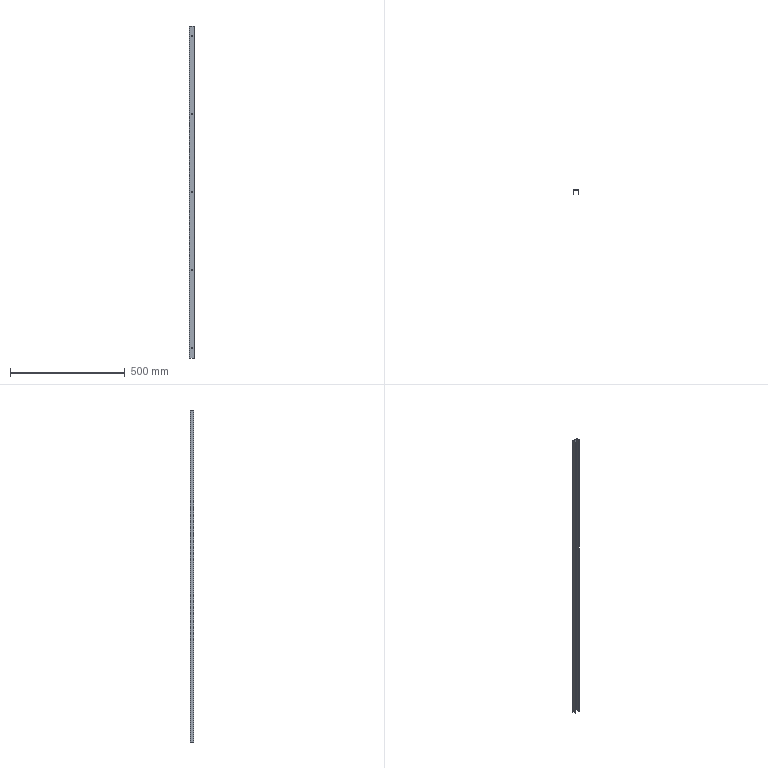Component | SolidWorks | GlassDoorAssembly-1_BentPlate-1 | 1 solid | 32 faces | box 25 x 16 x 1445 mm | volume 113630 mm3 | plane 18 | cylinder 14 | commonest cylinder face diameters 5.2 x10 5 x2 2 x2
STEP:
#1=CARTESIAN_POINT('',(-1.027,-19.472,-58.106));
#2=VERTEX_POINT('',#1);
#3=CARTESIAN_POINT('',(-1.027,-19.472,-58.311));
#4=VERTEX_POINT('',#3);
#5=CARTESIAN_POINT('',(-1.027,-19.472,-58.209));
#6=DIRECTION('',(0.,-1.,-0.));
#7=DIRECTION('',(0.,0.,-1.));
#8=AXIS2_PLACEMENT_3D('',#5,#6,#7);
#9=CIRCLE('',#8,0.1024);
#10=EDGE_CURVE('',#2,#4,#9,.T.);
#11=ORIENTED_EDGE('',*,*,#10,.T.);
#12=CARTESIAN_POINT('',(-1.027,-19.412,-58.311));
#13=VERTEX_POINT('',#12);
#14=CARTESIAN_POINT('',(-1.027,-19.491,-58.311));
#15=DIRECTION('',(-0.,1.,0.));
#16=VECTOR('',#15,39.37);
#17=LINE('',#14,#16);
#18=EDGE_CURVE('',#4,#13,#17,.T.);
#19=ORIENTED_EDGE('',*,*,#18,.T.);
#20=CARTESIAN_POINT('',(-1.027,-19.412,-58.106));
#21=VERTEX_POINT('',#20);
#22=CARTESIAN_POINT('',(-1.027,-19.412,-58.209));
#23=DIRECTION('',(-0.,1.,0.));
#24=DIRECTION('',(-0.,0.,1.));
#25=AXIS2_PLACEMENT_3D('',#22,#23,#24);
#26=CIRCLE('',#25,0.1024);
#27=EDGE_CURVE('',#13,#21,#26,.T.);
#28=ORIENTED_EDGE('',*,*,#27,.T.);
#29=CARTESIAN_POINT('',(-1.027,-19.491,-58.106));
#30=DIRECTION('',(-0.,1.,0.));
#31=VECTOR('',#30,39.37);
#32=LINE('',#29,#31);
#33=EDGE_CURVE('',#2,#21,#32,.T.);
#34=ORIENTED_EDGE('',*,*,#33,.F.);
#35=EDGE_LOOP('',(#11,#19,#28,#34));
#36=FACE_OUTER_BOUND('',#35,.T.);
#37=CARTESIAN_POINT('',(-1.027,-19.491,-58.209));
#38=DIRECTION('',(-0.,1.,0.));
#39=DIRECTION('',(-0.,0.,1.));
#40=AXIS2_PLACEMENT_3D('',#37,#38,#39);
#41=CYLINDRICAL_SURFACE('',#40,0.1024);
#42=ADVANCED_FACE('',(#36),#41,.F.);
#43=CARTESIAN_POINT('',(-1.027,-19.472,-44.72));
#44=VERTEX_POINT('',#43);
#45=CARTESIAN_POINT('',(-1.027,-19.472,-44.925));
#46=VERTEX_POINT('',#45);
#47=CARTESIAN_POINT('',(-1.027,-19.472,-44.823));
#48=DIRECTION('',(0.,-1.,-0.));
#49=DIRECTION('',(0.,0.,-1.));
#50=AXIS2_PLACEMENT_3D('',#47,#48,#49);
#51=CIRCLE('',#50,0.1024);
#52=EDGE_CURVE('',#44,#46,#51,.T.);
#53=ORIENTED_EDGE('',*,*,#52,.T.);
#54=CARTESIAN_POINT('',(-1.027,-19.412,-44.925));
#55=VERTEX_POINT('',#54);
#56=CARTESIAN_POINT('',(-1.027,-19.491,-44.925));
#57=DIRECTION('',(-0.,1.,0.));
#58=VECTOR('',#57,39.37);
#59=LINE('',#56,#58);
#60=EDGE_CURVE('',#46,#55,#59,.T.);
#61=ORIENTED_EDGE('',*,*,#60,.T.);
#62=CARTESIAN_POINT('',(-1.027,-19.412,-44.72));
#63=VERTEX_POINT('',#62);
#64=CARTESIAN_POINT('',(-1.027,-19.412,-44.823));
#65=DIRECTION('',(-0.,1.,0.));
#66=DIRECTION('',(-0.,0.,1.));
#67=AXIS2_PLACEMENT_3D('',#64,#65,#66);
#68=CIRCLE('',#67,0.1024);
#69=EDGE_CURVE('',#55,#63,#68,.T.);
#70=ORIENTED_EDGE('',*,*,#69,.T.);
#71=CARTESIAN_POINT('',(-1.027,-19.491,-44.72));
#72=DIRECTION('',(-0.,1.,0.));
#73=VECTOR('',#72,39.37);
#74=LINE('',#71,#73);
#75=EDGE_CURVE('',#44,#63,#74,.T.);
#76=ORIENTED_EDGE('',*,*,#75,.F.);
#77=EDGE_LOOP('',(#53,#61,#70,#76));
#78=FACE_OUTER_BOUND('',#77,.T.);
#79=CARTESIAN_POINT('',(-1.027,-19.491,-44.823));
#80=DIRECTION('',(-0.,1.,0.));
#81=DIRECTION('',(-0.,0.,1.));
#82=AXIS2_PLACEMENT_3D('',#79,#80,#81);
#83=CYLINDRICAL_SURFACE('',#82,0.1024);
#84=ADVANCED_FACE('',(#78),#83,.F.);
#85=CARTESIAN_POINT('',(-1.027,-19.472,-4.563));
#86=VERTEX_POINT('',#85);
#87=CARTESIAN_POINT('',(-1.027,-19.472,-4.768));
#88=VERTEX_POINT('',#87);
#89=CARTESIAN_POINT('',(-1.027,-19.472,-4.665));
#90=DIRECTION('',(0.,-1.,-0.));
#91=DIRECTION('',(0.,0.,-1.));
#92=AXIS2_PLACEMENT_3D('',#89,#90,#91);
#93=CIRCLE('',#92,0.1024);
#94=EDGE_CURVE('',#86,#88,#93,.T.);
#95=ORIENTED_EDGE('',*,*,#94,.T.);
#96=CARTESIAN_POINT('',(-1.027,-19.412,-4.768));
#97=VERTEX_POINT('',#96);
#98=CARTESIAN_POINT('',(-1.027,-19.491,-4.768));
#99=DIRECTION('',(-0.,1.,0.));
#100=VECTOR('',#99,39.37);
#101=LINE('',#98,#100);
#102=EDGE_CURVE('',#88,#97,#101,.T.);
#103=ORIENTED_EDGE('',*,*,#102,.T.);
#104=CARTESIAN_POINT('',(-1.027,-19.412,-4.563));
#105=VERTEX_POINT('',#104);
#106=CARTESIAN_POINT('',(-1.027,-19.412,-4.665));
#107=DIRECTION('',(-0.,1.,0.));
#108=DIRECTION('',(-0.,0.,1.));
#109=AXIS2_PLACEMENT_3D('',#106,#107,#108);
#110=CIRCLE('',#109,0.1024);
#111=EDGE_CURVE('',#97,#105,#110,.T.);
#112=ORIENTED_EDGE('',*,*,#111,.T.);
#113=CARTESIAN_POINT('',(-1.027,-19.491,-4.563));
#114=DIRECTION('',(-0.,1.,0.));
#115=VECTOR('',#114,39.37);
#116=LINE('',#113,#115);
#117=EDGE_CURVE('',#86,#105,#116,.T.);
#118=ORIENTED_EDGE('',*,*,#117,.F.);
#119=EDGE_LOOP('',(#95,#103,#112,#118));
#120=FACE_OUTER_BOUND('',#119,.T.);
#121=CARTESIAN_POINT('',(-1.027,-19.491,-4.665));
#122=DIRECTION('',(-0.,1.,0.));
#123=DIRECTION('',(-0.,0.,1.));
#124=AXIS2_PLACEMENT_3D('',#121,#122,#123);
#125=CYLINDRICAL_SURFACE('',#124,0.1024);
#126=ADVANCED_FACE('',(#120),#125,.F.);
#127=CARTESIAN_POINT('',(-1.027,-19.472,-17.949));
#128=VERTEX_POINT('',#127);
#129=CARTESIAN_POINT('',(-1.027,-19.472,-18.154));
#130=VERTEX_POINT('',#129);
#131=CARTESIAN_POINT('',(-1.027,-19.472,-18.051));
#132=DIRECTION('',(0.,-1.,-0.));
#133=DIRECTION('',(0.,0.,-1.));
#134=AXIS2_PLACEMENT_3D('',#131,#132,#133);
#135=CIRCLE('',#134,0.1024);
#136=EDGE_CURVE('',#128,#130,#135,.T.);
#137=ORIENTED_EDGE('',*,*,#136,.T.);
#138=CARTESIAN_POINT('',(-1.027,-19.412,-18.154));
#139=VERTEX_POINT('',#138);
#140=CARTESIAN_POINT('',(-1.027,-19.491,-18.154));
#141=DIRECTION('',(-0.,1.,0.));
#142=VECTOR('',#141,39.37);
#143=LINE('',#140,#142);
#144=EDGE_CURVE('',#130,#139,#143,.T.);
#145=ORIENTED_EDGE('',*,*,#144,.T.);
#146=CARTESIAN_POINT('',(-1.027,-19.412,-17.949));
#147=VERTEX_POINT('',#146);
#148=CARTESIAN_POINT('',(-1.027,-19.412,-18.051));
#149=DIRECTION('',(-0.,1.,0.));
#150=DIRECTION('',(-0.,0.,1.));
#151=AXIS2_PLACEMENT_3D('',#148,#149,#150);
#152=CIRCLE('',#151,0.1024);
#153=EDGE_CURVE('',#139,#147,#152,.T.);
#154=ORIENTED_EDGE('',*,*,#153,.T.);
#155=CARTESIAN_POINT('',(-1.027,-19.491,-17.949));
#156=DIRECTION('',(-0.,1.,0.));
#157=VECTOR('',#156,39.37);
#158=LINE('',#155,#157);
#159=EDGE_CURVE('',#128,#147,#158,.T.);
#160=ORIENTED_EDGE('',*,*,#159,.F.);
#161=EDGE_LOOP('',(#137,#145,#154,#160));
#162=FACE_OUTER_BOUND('',#161,.T.);
#163=CARTESIAN_POINT('',(-1.027,-19.491,-18.051));
#164=DIRECTION('',(-0.,1.,0.));
#165=DIRECTION('',(-0.,0.,1.));
#166=AXIS2_PLACEMENT_3D('',#163,#164,#165);
#167=CYLINDRICAL_SURFACE('',#166,0.1024);
#168=ADVANCED_FACE('',(#162),#167,.F.);
#169=CARTESIAN_POINT('',(-1.027,-19.472,-31.335));
#170=VERTEX_POINT('',#169);
#171=CARTESIAN_POINT('',(-1.027,-19.472,-31.539));
#172=VERTEX_POINT('',#171);
#173=CARTESIAN_POINT('',(-1.027,-19.472,-31.437));
#174=DIRECTION('',(0.,-1.,-0.));
#175=DIRECTION('',(0.,0.,-1.));
#176=AXIS2_PLACEMENT_3D('',#173,#174,#175);
#177=CIRCLE('',#176,0.1024);
#178=EDGE_CURVE('',#170,#172,#177,.T.);
#179=ORIENTED_EDGE('',*,*,#178,.T.);
#180=CARTESIAN_POINT('',(-1.027,-19.412,-31.539));
#181=VERTEX_POINT('',#180);
#182=CARTESIAN_POINT('',(-1.027,-19.491,-31.539));
#183=DIRECTION('',(-0.,1.,0.));
#184=VECTOR('',#183,39.37);
#185=LINE('',#182,#184);
#186=EDGE_CURVE('',#172,#181,#185,.T.);
#187=ORIENTED_EDGE('',*,*,#186,.T.);
#188=CARTESIAN_POINT('',(-1.027,-19.412,-31.335));
#189=VERTEX_POINT('',#188);
#190=CARTESIAN_POINT('',(-1.027,-19.412,-31.437));
#191=DIRECTION('',(-0.,1.,0.));
#192=DIRECTION('',(-0.,0.,1.));
#193=AXIS2_PLACEMENT_3D('',#190,#191,#192);
#194=CIRCLE('',#193,0.1024);
#195=EDGE_CURVE('',#181,#189,#194,.T.);
#196=ORIENTED_EDGE('',*,*,#195,.T.);
#197=CARTESIAN_POINT('',(-1.027,-19.491,-31.335));
#198=DIRECTION('',(-0.,1.,0.));
#199=VECTOR('',#198,39.37);
#200=LINE('',#197,#199);
#201=EDGE_CURVE('',#170,#189,#200,.T.);
#202=ORIENTED_EDGE('',*,*,#201,.F.);
#203=EDGE_LOOP('',(#179,#187,#196,#202));
#204=FACE_OUTER_BOUND('',#203,.T.);
#205=CARTESIAN_POINT('',(-1.027,-19.491,-31.437));
#206=DIRECTION('',(-0.,1.,0.));
#207=DIRECTION('',(-0.,0.,1.));
#208=AXIS2_PLACEMENT_3D('',#205,#206,#207);
#209=CYLINDRICAL_SURFACE('',#208,0.1024);
#210=ADVANCED_FACE('',(#204),#209,.F.);
#211=CARTESIAN_POINT('',(-1.027,-19.412,-58.209));
#212=DIRECTION('',(-0.,1.,0.));
#213=DIRECTION('',(-0.,0.,1.));
#214=AXIS2_PLACEMENT_3D('',#211,#212,#213);
#215=CIRCLE('',#214,0.1024);
#216=EDGE_CURVE('',#21,#13,#215,.T.);
#217=ORIENTED_EDGE('',*,*,#216,.F.);
#218=ORIENTED_EDGE('',*,*,#27,.F.);
#219=EDGE_LOOP('',(#217,#218));
#220=FACE_BOUND('',#219,.T.);
#221=CARTESIAN_POINT('',(-1.027,-19.412,-44.823));
#222=DIRECTION('',(-0.,1.,0.));
#223=DIRECTION('',(-0.,0.,1.));
#224=AXIS2_PLACEMENT_3D('',#221,#222,#223);
#225=CIRCLE('',#224,0.1024);
#226=EDGE_CURVE('',#63,#55,#225,.T.);
#227=ORIENTED_EDGE('',*,*,#226,.F.);
#228=ORIENTED_EDGE('',*,*,#69,.F.);
#229=EDGE_LOOP('',(#227,#228));
#230=FACE_BOUND('',#229,.T.);
#231=CARTESIAN_POINT('',(-1.027,-19.412,-4.665));
#232=DIRECTION('',(-0.,1.,0.));
#233=DIRECTION('',(-0.,0.,1.));
#234=AXIS2_PLACEMENT_3D('',#231,#232,#233);
#235=CIRCLE('',#234,0.1024);
#236=EDGE_CURVE('',#105,#97,#235,.T.);
#237=ORIENTED_EDGE('',*,*,#236,.F.);
#238=ORIENTED_EDGE('',*,*,#111,.F.);
#239=EDGE_LOOP('',(#237,#238));
#240=FACE_BOUND('',#239,.T.);
#241=CARTESIAN_POINT('',(-1.027,-19.412,-18.051));
#242=DIRECTION('',(-0.,1.,0.));
#243=DIRECTION('',(-0.,0.,1.));
#244=AXIS2_PLACEMENT_3D('',#241,#242,#243);
#245=CIRCLE('',#244,0.1024);
#246=EDGE_CURVE('',#147,#139,#245,.T.);
#247=ORIENTED_EDGE('',*,*,#246,.F.);
#248=ORIENTED_EDGE('',*,*,#153,.F.);
#249=EDGE_LOOP('',(#247,#248));
#250=FACE_BOUND('',#249,.T.);
#251=CARTESIAN_POINT('',(-1.027,-19.412,-31.437));
#252=DIRECTION('',(-0.,1.,0.));
#253=DIRECTION('',(-0.,0.,1.));
#254=AXIS2_PLACEMENT_3D('',#251,#252,#253);
#255=CIRCLE('',#254,0.1024);
#256=EDGE_CURVE('',#189,#181,#255,.T.);
#257=ORIENTED_EDGE('',*,*,#256,.F.);
#258=ORIENTED_EDGE('',*,*,#195,.F.);
#259=EDGE_LOOP('',(#257,#258));
#260=FACE_BOUND('',#259,.T.);
#261=CARTESIAN_POINT('',(-0.6329,-19.412,-2.992));
#262=VERTEX_POINT('',#261);
#263=CARTESIAN_POINT('',(-0.6329,-19.412,-59.882));
#264=VERTEX_POINT('',#263);
#265=CARTESIAN_POINT('',(-0.6329,-19.412,-2.992));
#266=DIRECTION('',(0.,0.,-1.));
#267=VECTOR('',#266,39.37);
#268=LINE('',#265,#267);
#269=EDGE_CURVE('',#262,#264,#268,.T.);
#270=ORIENTED_EDGE('',*,*,#269,.T.);
#271=CARTESIAN_POINT('',(-1.42,-19.412,-59.882));
#272=VERTEX_POINT('',#271);
#273=CARTESIAN_POINT('',(-0.5345,-19.412,-59.882));
#274=DIRECTION('',(1.,0.,0.));
#275=VECTOR('',#274,39.37);
#276=LINE('',#273,#275);
#277=EDGE_CURVE('',#272,#264,#276,.T.);
#278=ORIENTED_EDGE('',*,*,#277,.F.);
#279=CARTESIAN_POINT('',(-1.42,-19.412,-2.992));
#280=VERTEX_POINT('',#279);
#281=CARTESIAN_POINT('',(-1.42,-19.412,-59.882));
#282=DIRECTION('',(-0.,-0.,1.));
#283=VECTOR('',#282,39.37);
#284=LINE('',#281,#283);
#285=EDGE_CURVE('',#272,#280,#284,.T.);
#286=ORIENTED_EDGE('',*,*,#285,.T.);
#287=CARTESIAN_POINT('',(-0.5345,-19.412,-2.992));
#288=DIRECTION('',(-1.,-0.,-0.));
#289=VECTOR('',#288,39.37);
#290=LINE('',#287,#289);
#291=EDGE_CURVE('',#262,#280,#290,.T.);
#292=ORIENTED_EDGE('',*,*,#291,.F.);
#293=EDGE_LOOP('',(#270,#278,#286,#292));
#294=FACE_OUTER_BOUND('',#293,.T.);
#295=CARTESIAN_POINT('',(-1.519,-19.412,-59.882));
#296=DIRECTION('',(0.,-1.,-0.));
#297=DIRECTION('',(0.,0.,-1.));
#298=AXIS2_PLACEMENT_3D('',#295,#296,#297);
#299=PLANE('',#298);
#300=ADVANCED_FACE('',(#220,#230,#240,#250,#260,#294),#299,.F.);
#301=ORIENTED_EDGE('',*,*,#10,.F.);
#302=CARTESIAN_POINT('',(-1.027,-19.472,-58.209));
#303=DIRECTION('',(0.,-1.,-0.));
#304=DIRECTION('',(0.,0.,-1.));
#305=AXIS2_PLACEMENT_3D('',#302,#303,#304);
#306=CIRCLE('',#305,0.1024);
#307=EDGE_CURVE('',#4,#2,#306,.T.);
#308=ORIENTED_EDGE('',*,*,#307,.F.);
#309=EDGE_LOOP('',(#301,#308));
#310=FACE_BOUND('',#309,.T.);
#311=ORIENTED_EDGE('',*,*,#52,.F.);
#312=CARTESIAN_POINT('',(-1.027,-19.472,-44.823));
#313=DIRECTION('',(0.,-1.,-0.));
#314=DIRECTION('',(0.,0.,-1.));
#315=AXIS2_PLACEMENT_3D('',#312,#313,#314);
#316=CIRCLE('',#315,0.1024);
#317=EDGE_CURVE('',#46,#44,#316,.T.);
#318=ORIENTED_EDGE('',*,*,#317,.F.);
#319=EDGE_LOOP('',(#311,#318));
#320=FACE_BOUND('',#319,.T.);
#321=ORIENTED_EDGE('',*,*,#94,.F.);
#322=CARTESIAN_POINT('',(-1.027,-19.472,-4.665));
#323=DIRECTION('',(0.,-1.,-0.));
#324=DIRECTION('',(0.,0.,-1.));
#325=AXIS2_PLACEMENT_3D('',#322,#323,#324);
#326=CIRCLE('',#325,0.1024);
#327=EDGE_CURVE('',#88,#86,#326,.T.);
#328=ORIENTED_EDGE('',*,*,#327,.F.);
#329=EDGE_LOOP('',(#321,#328));
#330=FACE_BOUND('',#329,.T.);
#331=ORIENTED_EDGE('',*,*,#136,.F.);
#332=CARTESIAN_POINT('',(-1.027,-19.472,-18.051));
#333=DIRECTION('',(0.,-1.,-0.));
#334=DIRECTION('',(0.,0.,-1.));
#335=AXIS2_PLACEMENT_3D('',#332,#333,#334);
#336=CIRCLE('',#335,0.1024);
#337=EDGE_CURVE('',#130,#128,#336,.T.);
#338=ORIENTED_EDGE('',*,*,#337,.F.);
#339=EDGE_LOOP('',(#331,#338));
#340=FACE_BOUND('',#339,.T.);
#341=ORIENTED_EDGE('',*,*,#178,.F.);
#342=CARTESIAN_POINT('',(-1.027,-19.472,-31.437));
#343=DIRECTION('',(0.,-1.,-0.));
#344=DIRECTION('',(0.,0.,-1.));
#345=AXIS2_PLACEMENT_3D('',#342,#343,#344);
#346=CIRCLE('',#345,0.1024);
#347=EDGE_CURVE('',#172,#170,#346,.T.);
#348=ORIENTED_EDGE('',*,*,#347,.F.);
#349=EDGE_LOOP('',(#341,#348));
#350=FACE_BOUND('',#349,.T.);
#351=CARTESIAN_POINT('',(-1.42,-19.472,-59.882));
#352=VERTEX_POINT('',#351);
#353=CARTESIAN_POINT('',(-0.6329,-19.472,-59.882));
#354=VERTEX_POINT('',#353);
#355=CARTESIAN_POINT('',(-0.5345,-19.472,-59.882));
#356=DIRECTION('',(1.,0.,0.));
#357=VECTOR('',#356,39.37);
#358=LINE('',#355,#357);
#359=EDGE_CURVE('',#352,#354,#358,.T.);
#360=ORIENTED_EDGE('',*,*,#359,.T.);
#361=CARTESIAN_POINT('',(-0.6329,-19.472,-2.992));
#362=VERTEX_POINT('',#361);
#363=CARTESIAN_POINT('',(-0.6329,-19.472,-2.992));
#364=DIRECTION('',(0.,0.,-1.));
#365=VECTOR('',#364,39.37);
#366=LINE('',#363,#365);
#367=EDGE_CURVE('',#362,#354,#366,.T.);
#368=ORIENTED_EDGE('',*,*,#367,.F.);
#369=CARTESIAN_POINT('',(-1.42,-19.472,-2.992));
#370=VERTEX_POINT('',#369);
#371=CARTESIAN_POINT('',(-0.5345,-19.472,-2.992));
#372=DIRECTION('',(-1.,-0.,-0.));
#373=VECTOR('',#372,39.37);
#374=LINE('',#371,#373);
#375=EDGE_CURVE('',#362,#370,#374,.T.);
#376=ORIENTED_EDGE('',*,*,#375,.T.);
#377=CARTESIAN_POINT('',(-1.42,-19.472,-59.882));
#378=DIRECTION('',(-0.,-0.,1.));
#379=VECTOR('',#378,39.37);
#380=LINE('',#377,#379);
#381=EDGE_CURVE('',#352,#370,#380,.T.);
#382=ORIENTED_EDGE('',*,*,#381,.F.);
#383=EDGE_LOOP('',(#360,#368,#376,#382));
#384=FACE_OUTER_BOUND('',#383,.T.);
#385=CARTESIAN_POINT('',(-1.519,-19.472,-59.882));
#386=DIRECTION('',(0.,-1.,-0.));
#387=DIRECTION('',(0.,0.,-1.));
#388=AXIS2_PLACEMENT_3D('',#385,#386,#387);
#389=PLANE('',#388);
#390=ADVANCED_FACE('',(#310,#320,#330,#340,#350,#384),#389,.T.);
#391=ORIENTED_EDGE('',*,*,#375,.F.);
#392=CARTESIAN_POINT('',(-0.6329,-19.472,-2.992));
#393=DIRECTION('',(-0.,1.,0.));
#394=VECTOR('',#393,39.37);
#395=LINE('',#392,#394);
#396=EDGE_CURVE('',#362,#262,#395,.T.);
#397=ORIENTED_EDGE('',*,*,#396,.T.);
#398=ORIENTED_EDGE('',*,*,#291,.T.);
#399=CARTESIAN_POINT('',(-1.42,-19.472,-2.992));
#400=DIRECTION('',(-0.,1.,0.));
#401=VECTOR('',#400,39.37);
#402=LINE('',#399,#401);
#403=EDGE_CURVE('',#370,#280,#402,.T.);
#404=ORIENTED_EDGE('',*,*,#403,.F.);
#405=EDGE_LOOP('',(#391,#397,#398,#404));
#406=FACE_OUTER_BOUND('',#405,.T.);
#407=CARTESIAN_POINT('',(-0.5345,-19.412,-2.992));
#408=DIRECTION('',(-0.,-0.,1.));
#409=DIRECTION('',(0.,-1.,-0.));
#410=AXIS2_PLACEMENT_3D('',#407,#408,#409);
#411=PLANE('',#410);
#412=ADVANCED_FACE('',(#406),#411,.T.);
#413=CARTESIAN_POINT('',(-0.6329,-19.472,-59.882));
#414=DIRECTION('',(-0.,1.,0.));
#415=VECTOR('',#414,39.37);
#416=LINE('',#413,#415);
#417=EDGE_CURVE('',#354,#264,#416,.T.);
#418=ORIENTED_EDGE('',*,*,#417,.F.);
#419=ORIENTED_EDGE('',*,*,#359,.F.);
#420=CARTESIAN_POINT('',(-1.42,-19.472,-59.882));
#421=DIRECTION('',(-0.,1.,0.));
#422=VECTOR('',#421,39.37);
#423=LINE('',#420,#422);
#424=EDGE_CURVE('',#352,#272,#423,.T.);
#425=ORIENTED_EDGE('',*,*,#424,.T.);
#426=ORIENTED_EDGE('',*,*,#277,.T.);
#427=EDGE_LOOP('',(#418,#419,#425,#426));
#428=FACE_OUTER_BOUND('',#427,.T.);
#429=CARTESIAN_POINT('',(-0.5345,-19.412,-59.882));
#430=DIRECTION('',(0.,0.,-1.));
#431=DIRECTION('',(-0.,1.,0.));
#432=AXIS2_PLACEMENT_3D('',#429,#430,#431);
#433=PLANE('',#432);
#434=ADVANCED_FACE('',(#428),#433,.T.);
#435=CARTESIAN_POINT('',(-1.46,-19.511,-2.992));
#436=VERTEX_POINT('',#435);
#437=CARTESIAN_POINT('',(-1.519,-19.511,-2.992));
#438=VERTEX_POINT('',#437);
#439=CARTESIAN_POINT('',(-1.519,-19.511,-2.992));
#440=DIRECTION('',(-1.,-0.,-0.));
#441=VECTOR('',#440,39.37);
#442=LINE('',#439,#441);
#443=EDGE_CURVE('',#436,#438,#442,.T.);
#444=ORIENTED_EDGE('',*,*,#443,.F.);
#445=CARTESIAN_POINT('',(-1.42,-19.511,-2.992));
#446=DIRECTION('',(-0.,-0.,1.));
#447=DIRECTION('',(0.,1.,0.));
#448=AXIS2_PLACEMENT_3D('',#445,#446,#447);
#449=CIRCLE('',#448,0.03937);
#450=EDGE_CURVE('',#370,#436,#449,.T.);
#451=ORIENTED_EDGE('',*,*,#450,.F.);
#452=ORIENTED_EDGE('',*,*,#403,.T.);
#453=CARTESIAN_POINT('',(-1.42,-19.511,-2.992));
#454=DIRECTION('',(-0.,-0.,1.));
#455=DIRECTION('',(-0.,1.,0.));
#456=AXIS2_PLACEMENT_3D('',#453,#454,#455);
#457=CIRCLE('',#456,0.09843);
#458=EDGE_CURVE('',#280,#438,#457,.T.);
#459=ORIENTED_EDGE('',*,*,#458,.T.);
#460=EDGE_LOOP('',(#444,#451,#452,#459));
#461=FACE_OUTER_BOUND('',#460,.T.);
#462=CARTESIAN_POINT('',(-1.42,-19.511,-2.992));
#463=DIRECTION('',(-0.,-0.,1.));
#464=DIRECTION('',(0.,-1.,-0.));
#465=AXIS2_PLACEMENT_3D('',#462,#463,#464);
#466=PLANE('',#465);
#467=ADVANCED_FACE('',(#461),#466,.T.);
#468=CARTESIAN_POINT('',(-1.46,-19.511,-59.882));
#469=VERTEX_POINT('',#468);
#470=CARTESIAN_POINT('',(-1.42,-19.511,-59.882));
#471=DIRECTION('',(0.,0.,-1.));
#472=DIRECTION('',(-0.,1.,0.));
#473=AXIS2_PLACEMENT_3D('',#470,#471,#472);
#474=CIRCLE('',#473,0.03937);
#475=EDGE_CURVE('',#469,#352,#474,.T.);
#476=ORIENTED_EDGE('',*,*,#475,.F.);
#477=CARTESIAN_POINT('',(-1.519,-19.511,-59.882));
#478=VERTEX_POINT('',#477);
#479=CARTESIAN_POINT('',(-1.46,-19.511,-59.882));
#480=DIRECTION('',(-1.,-0.,-0.));
#481=VECTOR('',#480,39.37);
#482=LINE('',#479,#481);
#483=EDGE_CURVE('',#469,#478,#482,.T.);
#484=ORIENTED_EDGE('',*,*,#483,.T.);
#485=CARTESIAN_POINT('',(-1.42,-19.511,-59.882));
#486=DIRECTION('',(0.,0.,-1.));
#487=DIRECTION('',(-0.,1.,0.));
#488=AXIS2_PLACEMENT_3D('',#485,#486,#487);
#489=CIRCLE('',#488,0.09843);
#490=EDGE_CURVE('',#478,#272,#489,.T.);
#491=ORIENTED_EDGE('',*,*,#490,.T.);
#492=ORIENTED_EDGE('',*,*,#424,.F.);
#493=EDGE_LOOP('',(#476,#484,#491,#492));
#494=FACE_OUTER_BOUND('',#493,.T.);
#495=CARTESIAN_POINT('',(-1.42,-19.511,-59.882));
#496=DIRECTION('',(-0.,-0.,1.));
#497=DIRECTION('',(0.,-1.,-0.));
#498=AXIS2_PLACEMENT_3D('',#495,#496,#497);
#499=PLANE('',#498);
#500=ADVANCED_FACE('',(#494),#499,.F.);
#501=ORIENTED_EDGE('',*,*,#285,.F.);
#502=ORIENTED_EDGE('',*,*,#490,.F.);
#503=CARTESIAN_POINT('',(-1.519,-19.511,-2.992));
#504=DIRECTION('',(-0.,-0.,1.));
#505=VECTOR('',#504,39.37);
#506=LINE('',#503,#505);
#507=EDGE_CURVE('',#478,#438,#506,.T.);
#508=ORIENTED_EDGE('',*,*,#507,.T.);
#509=ORIENTED_EDGE('',*,*,#458,.F.);
#510=EDGE_LOOP('',(#501,#502,#508,#509));
#511=FACE_OUTER_BOUND('',#510,.T.);
#512=CARTESIAN_POINT('',(-1.42,-19.511,-59.882));
#513=DIRECTION('',(0.,0.,-1.));
#514=DIRECTION('',(-1.,0.,0.));
#515=AXIS2_PLACEMENT_3D('',#512,#513,#514);
#516=CYLINDRICAL_SURFACE('',#515,0.09843);
#517=ADVANCED_FACE('',(#511),#516,.T.);
#518=ORIENTED_EDGE('',*,*,#381,.T.);
#519=ORIENTED_EDGE('',*,*,#450,.T.);
#520=CARTESIAN_POINT('',(-1.46,-19.511,-2.992));
#521=DIRECTION('',(0.,0.,-1.));
#522=VECTOR('',#521,39.37);
#523=LINE('',#520,#522);
#524=EDGE_CURVE('',#436,#469,#523,.T.);
#525=ORIENTED_EDGE('',*,*,#524,.T.);
#526=ORIENTED_EDGE('',*,*,#475,.T.);
#527=EDGE_LOOP('',(#518,#519,#525,#526));
#528=FACE_OUTER_BOUND('',#527,.T.);
#529=CARTESIAN_POINT('',(-1.42,-19.511,-59.882));
#530=DIRECTION('',(0.,0.,-1.));
#531=DIRECTION('',(-1.,0.,0.));
#532=AXIS2_PLACEMENT_3D('',#529,#530,#531);
#533=CYLINDRICAL_SURFACE('',#532,0.03937);
#534=ADVANCED_FACE('',(#528),#533,.F.);
#535=ORIENTED_EDGE('',*,*,#443,.T.);
#536=CARTESIAN_POINT('',(-1.519,-20.042,-2.992));
#537=VERTEX_POINT('',#536);
#538=CARTESIAN_POINT('',(-1.519,-20.042,-2.992));
#539=DIRECTION('',(-0.,1.,0.));
#540=VECTOR('',#539,39.37);
#541=LINE('',#538,#540);
#542=EDGE_CURVE('',#537,#438,#541,.T.);
#543=ORIENTED_EDGE('',*,*,#542,.F.);
#544=CARTESIAN_POINT('',(-1.46,-20.042,-2.992));
#545=VERTEX_POINT('',#544);
#546=CARTESIAN_POINT('',(-1.519,-20.042,-2.992));
#547=DIRECTION('',(1.,0.,0.));
#548=VECTOR('',#547,39.37);
#549=LINE('',#546,#548);
#550=EDGE_CURVE('',#537,#545,#549,.T.);
#551=ORIENTED_EDGE('',*,*,#550,.T.);
#552=CARTESIAN_POINT('',(-1.46,-19.472,-2.992));
#553=DIRECTION('',(-0.,1.,0.));
#554=VECTOR('',#553,39.37);
#555=LINE('',#552,#554);
#556=EDGE_CURVE('',#545,#436,#555,.T.);
#557=ORIENTED_EDGE('',*,*,#556,.T.);
#558=EDGE_LOOP('',(#535,#543,#551,#557));
#559=FACE_OUTER_BOUND('',#558,.T.);
#560=CARTESIAN_POINT('',(-1.519,-19.472,-2.992));
#561=DIRECTION('',(0.,0.,-1.));
#562=DIRECTION('',(-0.,1.,0.));
#563=AXIS2_PLACEMENT_3D('',#560,#561,#562);
#564=PLANE('',#563);
#565=ADVANCED_FACE('',(#559),#564,.F.);
#566=ORIENTED_EDGE('',*,*,#483,.F.);
#567=CARTESIAN_POINT('',(-1.46,-20.042,-59.882));
#568=VERTEX_POINT('',#567);
#569=CARTESIAN_POINT('',(-1.46,-20.042,-59.882));
#570=DIRECTION('',(0.,-1.,-0.));
#571=VECTOR('',#570,39.37);
#572=LINE('',#569,#571);
#573=EDGE_CURVE('',#469,#568,#572,.T.);
#574=ORIENTED_EDGE('',*,*,#573,.T.);
#575=CARTESIAN_POINT('',(-1.519,-20.042,-59.882));
#576=VERTEX_POINT('',#575);
#577=CARTESIAN_POINT('',(-1.519,-20.042,-59.882));
#578=DIRECTION('',(1.,0.,0.));
#579=VECTOR('',#578,39.37);
#580=LINE('',#577,#579);
#581=EDGE_CURVE('',#576,#568,#580,.T.);
#582=ORIENTED_EDGE('',*,*,#581,.F.);
#583=CARTESIAN_POINT('',(-1.519,-20.042,-59.882));
#584=DIRECTION('',(0.,-1.,-0.));
#585=VECTOR('',#584,39.37);
#586=LINE('',#583,#585);
#587=EDGE_CURVE('',#478,#576,#586,.T.);
#588=ORIENTED_EDGE('',*,*,#587,.F.);
#589=EDGE_LOOP('',(#566,#574,#582,#588));
#590=FACE_OUTER_BOUND('',#589,.T.);
#591=CARTESIAN_POINT('',(-1.519,-20.042,-59.882));
#592=DIRECTION('',(-0.,-0.,1.));
#593=DIRECTION('',(0.,-1.,-0.));
#594=AXIS2_PLACEMENT_3D('',#591,#592,#593);
#595=PLANE('',#594);
#596=ADVANCED_FACE('',(#590),#595,.F.);
#597=ORIENTED_EDGE('',*,*,#507,.F.);
#598=ORIENTED_EDGE('',*,*,#587,.T.);
#599=CARTESIAN_POINT('',(-1.519,-20.042,-2.992));
#600=DIRECTION('',(-0.,-0.,1.));
#601=VECTOR('',#600,39.37);
#602=LINE('',#599,#601);
#603=EDGE_CURVE('',#576,#537,#602,.T.);
#604=ORIENTED_EDGE('',*,*,#603,.T.);
#605=ORIENTED_EDGE('',*,*,#542,.T.);
#606=EDGE_LOOP('',(#597,#598,#604,#605));
#607=FACE_OUTER_BOUND('',#606,.T.);
#608=CARTESIAN_POINT('',(-1.519,-20.042,-2.992));
#609=DIRECTION('',(1.,0.,0.));
#610=DIRECTION('',(0.,-1.,-0.));
#611=AXIS2_PLACEMENT_3D('',#608,#609,#610);
#612=PLANE('',#611);
#613=ADVANCED_FACE('',(#607),#612,.F.);
#614=ORIENTED_EDGE('',*,*,#573,.F.);
#615=ORIENTED_EDGE('',*,*,#524,.F.);
#616=ORIENTED_EDGE('',*,*,#556,.F.);
#617=CARTESIAN_POINT('',(-1.46,-20.042,-2.992));
#618=DIRECTION('',(-0.,-0.,1.));
#619=VECTOR('',#618,39.37);
#620=LINE('',#617,#619);
#621=EDGE_CURVE('',#568,#545,#620,.T.);
#622=ORIENTED_EDGE('',*,*,#621,.F.);
#623=EDGE_LOOP('',(#614,#615,#616,#622));
#624=FACE_OUTER_BOUND('',#623,.T.);
#625=CARTESIAN_POINT('',(-1.46,-20.042,-2.992));
#626=DIRECTION('',(1.,0.,0.));
#627=DIRECTION('',(0.,-1.,-0.));
#628=AXIS2_PLACEMENT_3D('',#625,#626,#627);
#629=PLANE('',#628);
#630=ADVANCED_FACE('',(#624),#629,.T.);
#631=ORIENTED_EDGE('',*,*,#621,.T.);
#632=ORIENTED_EDGE('',*,*,#550,.F.);
#633=ORIENTED_EDGE('',*,*,#603,.F.);
#634=ORIENTED_EDGE('',*,*,#581,.T.);
#635=EDGE_LOOP('',(#631,#632,#633,#634));
#636=FACE_OUTER_BOUND('',#635,.T.);
#637=CARTESIAN_POINT('',(-1.519,-20.042,-2.992));
#638=DIRECTION('',(-0.,1.,0.));
#639=DIRECTION('',(1.,0.,0.));
#640=AXIS2_PLACEMENT_3D('',#637,#638,#639);
#641=PLANE('',#640);
#642=ADVANCED_FACE('',(#636),#641,.F.);
#643=CARTESIAN_POINT('',(-0.5936,-19.511,-59.882));
#644=VERTEX_POINT('',#643);
#645=CARTESIAN_POINT('',(-0.5345,-19.511,-59.882));
#646=VERTEX_POINT('',#645);
#647=CARTESIAN_POINT('',(-0.5345,-19.511,-59.882));
#648=DIRECTION('',(1.,0.,0.));
#649=VECTOR('',#648,39.37);
#650=LINE('',#647,#649);
#651=EDGE_CURVE('',#644,#646,#650,.T.);
#652=ORIENTED_EDGE('',*,*,#651,.F.);
#653=CARTESIAN_POINT('',(-0.6329,-19.511,-59.882));
#654=DIRECTION('',(0.,0.,-1.));
#655=DIRECTION('',(0.,-1.,0.));
#656=AXIS2_PLACEMENT_3D('',#653,#654,#655);
#657=CIRCLE('',#656,0.03937);
#658=EDGE_CURVE('',#354,#644,#657,.T.);
#659=ORIENTED_EDGE('',*,*,#658,.F.);
#660=ORIENTED_EDGE('',*,*,#417,.T.);
#661=CARTESIAN_POINT('',(-0.6329,-19.511,-59.882));
#662=DIRECTION('',(0.,0.,-1.));
#663=DIRECTION('',(0.,-1.,0.));
#664=AXIS2_PLACEMENT_3D('',#661,#662,#663);
#665=CIRCLE('',#664,0.09843);
#666=EDGE_CURVE('',#264,#646,#665,.T.);
#667=ORIENTED_EDGE('',*,*,#666,.T.);
#668=EDGE_LOOP('',(#652,#659,#660,#667));
#669=FACE_OUTER_BOUND('',#668,.T.);
#670=CARTESIAN_POINT('',(-0.6329,-19.511,-59.882));
#671=DIRECTION('',(0.,0.,-1.));
#672=DIRECTION('',(-0.,1.,0.));
#673=AXIS2_PLACEMENT_3D('',#670,#671,#672);
#674=PLANE('',#673);
#675=ADVANCED_FACE('',(#669),#674,.T.);
#676=CARTESIAN_POINT('',(-0.5936,-19.511,-2.992));
#677=VERTEX_POINT('',#676);
#678=CARTESIAN_POINT('',(-0.6329,-19.511,-2.992));
#679=DIRECTION('',(-0.,-0.,1.));
#680=DIRECTION('',(0.,-1.,0.));
#681=AXIS2_PLACEMENT_3D('',#678,#679,#680);
#682=CIRCLE('',#681,0.03937);
#683=EDGE_CURVE('',#677,#362,#682,.T.);
#684=ORIENTED_EDGE('',*,*,#683,.F.);
#685=CARTESIAN_POINT('',(-0.5345,-19.511,-2.992));
#686=VERTEX_POINT('',#685);
#687=CARTESIAN_POINT('',(-0.5936,-19.511,-2.992));
#688=DIRECTION('',(1.,0.,0.));
#689=VECTOR('',#688,39.37);
#690=LINE('',#687,#689);
#691=EDGE_CURVE('',#677,#686,#690,.T.);
#692=ORIENTED_EDGE('',*,*,#691,.T.);
#693=CARTESIAN_POINT('',(-0.6329,-19.511,-2.992));
#694=DIRECTION('',(-0.,-0.,1.));
#695=DIRECTION('',(0.,-1.,0.));
#696=AXIS2_PLACEMENT_3D('',#693,#694,#695);
#697=CIRCLE('',#696,0.09843);
#698=EDGE_CURVE('',#686,#262,#697,.T.);
#699=ORIENTED_EDGE('',*,*,#698,.T.);
#700=ORIENTED_EDGE('',*,*,#396,.F.);
#701=EDGE_LOOP('',(#684,#692,#699,#700));
#702=FACE_OUTER_BOUND('',#701,.T.);
#703=CARTESIAN_POINT('',(-0.6329,-19.511,-2.992));
#704=DIRECTION('',(0.,0.,-1.));
#705=DIRECTION('',(-0.,1.,0.));
#706=AXIS2_PLACEMENT_3D('',#703,#704,#705);
#707=PLANE('',#706);
#708=ADVANCED_FACE('',(#702),#707,.F.);
#709=ORIENTED_EDGE('',*,*,#269,.F.);
#710=ORIENTED_EDGE('',*,*,#698,.F.);
#711=CARTESIAN_POINT('',(-0.5345,-19.511,-59.882));
#712=DIRECTION('',(0.,0.,-1.));
#713=VECTOR('',#712,39.37);
#714=LINE('',#711,#713);
#715=EDGE_CURVE('',#686,#646,#714,.T.);
#716=ORIENTED_EDGE('',*,*,#715,.T.);
#717=ORIENTED_EDGE('',*,*,#666,.F.);
#718=EDGE_LOOP('',(#709,#710,#716,#717));
#719=FACE_OUTER_BOUND('',#718,.T.);
#720=CARTESIAN_POINT('',(-0.6329,-19.511,-2.992));
#721=DIRECTION('',(-0.,-0.,1.));
#722=DIRECTION('',(1.,0.,0.));
#723=AXIS2_PLACEMENT_3D('',#720,#721,#722);
#724=CYLINDRICAL_SURFACE('',#723,0.09843);
#725=ADVANCED_FACE('',(#719),#724,.T.);
#726=ORIENTED_EDGE('',*,*,#367,.T.);
#727=ORIENTED_EDGE('',*,*,#658,.T.);
#728=CARTESIAN_POINT('',(-0.5936,-19.511,-59.882));
#729=DIRECTION('',(-0.,-0.,1.));
#730=VECTOR('',#729,39.37);
#731=LINE('',#728,#730);
#732=EDGE_CURVE('',#644,#677,#731,.T.);
#733=ORIENTED_EDGE('',*,*,#732,.T.);
#734=ORIENTED_EDGE('',*,*,#683,.T.);
#735=EDGE_LOOP('',(#726,#727,#733,#734));
#736=FACE_OUTER_BOUND('',#735,.T.);
#737=CARTESIAN_POINT('',(-0.6329,-19.511,-2.992));
#738=DIRECTION('',(-0.,-0.,1.));
#739=DIRECTION('',(1.,0.,0.));
#740=AXIS2_PLACEMENT_3D('',#737,#738,#739);
#741=CYLINDRICAL_SURFACE('',#740,0.03937);
#742=ADVANCED_FACE('',(#736),#741,.F.);
#743=ORIENTED_EDGE('',*,*,#651,.T.);
#744=CARTESIAN_POINT('',(-0.5345,-20.042,-59.882));
#745=VERTEX_POINT('',#744);
#746=CARTESIAN_POINT('',(-0.5345,-20.042,-59.882));
#747=DIRECTION('',(-0.,1.,0.));
#748=VECTOR('',#747,39.37);
#749=LINE('',#746,#748);
#750=EDGE_CURVE('',#745,#646,#749,.T.);
#751=ORIENTED_EDGE('',*,*,#750,.F.);
#752=CARTESIAN_POINT('',(-0.5936,-20.042,-59.882));
#753=VERTEX_POINT('',#752);
#754=CARTESIAN_POINT('',(-0.5345,-20.042,-59.882));
#755=DIRECTION('',(-1.,-0.,-0.));
#756=VECTOR('',#755,39.37);
#757=LINE('',#754,#756);
#758=EDGE_CURVE('',#745,#753,#757,.T.);
#759=ORIENTED_EDGE('',*,*,#758,.T.);
#760=CARTESIAN_POINT('',(-0.5936,-19.472,-59.882));
#761=DIRECTION('',(-0.,1.,0.));
#762=VECTOR('',#761,39.37);
#763=LINE('',#760,#762);
#764=EDGE_CURVE('',#753,#644,#763,.T.);
#765=ORIENTED_EDGE('',*,*,#764,.T.);
#766=EDGE_LOOP('',(#743,#751,#759,#765));
#767=FACE_OUTER_BOUND('',#766,.T.);
#768=CARTESIAN_POINT('',(-0.5345,-19.472,-59.882));
#769=DIRECTION('',(-0.,-0.,1.));
#770=DIRECTION('',(0.,-1.,-0.));
#771=AXIS2_PLACEMENT_3D('',#768,#769,#770);
#772=PLANE('',#771);
#773=ADVANCED_FACE('',(#767),#772,.F.);
#774=ORIENTED_EDGE('',*,*,#691,.F.);
#775=CARTESIAN_POINT('',(-0.5936,-20.042,-2.992));
#776=VERTEX_POINT('',#775);
#777=CARTESIAN_POINT('',(-0.5936,-20.042,-2.992));
#778=DIRECTION('',(0.,-1.,-0.));
#779=VECTOR('',#778,39.37);
#780=LINE('',#777,#779);
#781=EDGE_CURVE('',#677,#776,#780,.T.);
#782=ORIENTED_EDGE('',*,*,#781,.T.);
#783=CARTESIAN_POINT('',(-0.5345,-20.042,-2.992));
#784=VERTEX_POINT('',#783);
#785=CARTESIAN_POINT('',(-0.5345,-20.042,-2.992));
#786=DIRECTION('',(-1.,-0.,-0.));
#787=VECTOR('',#786,39.37);
#788=LINE('',#785,#787);
#789=EDGE_CURVE('',#784,#776,#788,.T.);
#790=ORIENTED_EDGE('',*,*,#789,.F.);
#791=CARTESIAN_POINT('',(-0.5345,-20.042,-2.992));
#792=DIRECTION('',(0.,-1.,-0.));
#793=VECTOR('',#792,39.37);
#794=LINE('',#791,#793);
#795=EDGE_CURVE('',#686,#784,#794,.T.);
#796=ORIENTED_EDGE('',*,*,#795,.F.);
#797=EDGE_LOOP('',(#774,#782,#790,#796));
#798=FACE_OUTER_BOUND('',#797,.T.);
#799=CARTESIAN_POINT('',(-0.5345,-20.042,-2.992));
#800=DIRECTION('',(0.,0.,-1.));
#801=DIRECTION('',(-0.,1.,0.));
#802=AXIS2_PLACEMENT_3D('',#799,#800,#801);
#803=PLANE('',#802);
#804=ADVANCED_FACE('',(#798),#803,.F.);
#805=ORIENTED_EDGE('',*,*,#715,.F.);
#806=ORIENTED_EDGE('',*,*,#795,.T.);
#807=CARTESIAN_POINT('',(-0.5345,-20.042,-59.882));
#808=DIRECTION('',(0.,0.,-1.));
#809=VECTOR('',#808,39.37);
#810=LINE('',#807,#809);
#811=EDGE_CURVE('',#784,#745,#810,.T.);
#812=ORIENTED_EDGE('',*,*,#811,.T.);
#813=ORIENTED_EDGE('',*,*,#750,.T.);
#814=EDGE_LOOP('',(#805,#806,#812,#813));
#815=FACE_OUTER_BOUND('',#814,.T.);
#816=CARTESIAN_POINT('',(-0.5345,-20.042,-59.882));
#817=DIRECTION('',(-1.,-0.,-0.));
#818=DIRECTION('',(-0.,1.,0.));
#819=AXIS2_PLACEMENT_3D('',#816,#817,#818);
#820=PLANE('',#819);
#821=ADVANCED_FACE('',(#815),#820,.F.);
#822=ORIENTED_EDGE('',*,*,#781,.F.);
#823=ORIENTED_EDGE('',*,*,#732,.F.);
#824=ORIENTED_EDGE('',*,*,#764,.F.);
#825=CARTESIAN_POINT('',(-0.5936,-20.042,-59.882));
#826=DIRECTION('',(0.,0.,-1.));
#827=VECTOR('',#826,39.37);
#828=LINE('',#825,#827);
#829=EDGE_CURVE('',#776,#753,#828,.T.);
#830=ORIENTED_EDGE('',*,*,#829,.F.);
#831=EDGE_LOOP('',(#822,#823,#824,#830));
#832=FACE_OUTER_BOUND('',#831,.T.);
#833=CARTESIAN_POINT('',(-0.5936,-20.042,-59.882));
#834=DIRECTION('',(-1.,-0.,-0.));
#835=DIRECTION('',(-0.,1.,0.));
#836=AXIS2_PLACEMENT_3D('',#833,#834,#835);
#837=PLANE('',#836);
#838=ADVANCED_FACE('',(#832),#837,.T.);
#839=ORIENTED_EDGE('',*,*,#829,.T.);
#840=ORIENTED_EDGE('',*,*,#758,.F.);
#841=ORIENTED_EDGE('',*,*,#811,.F.);
#842=ORIENTED_EDGE('',*,*,#789,.T.);
#843=EDGE_LOOP('',(#839,#840,#841,#842));
#844=FACE_OUTER_BOUND('',#843,.T.);
#845=CARTESIAN_POINT('',(-0.5345,-20.042,-59.882));
#846=DIRECTION('',(-0.,1.,0.));
#847=DIRECTION('',(1.,0.,0.));
#848=AXIS2_PLACEMENT_3D('',#845,#846,#847);
#849=PLANE('',#848);
#850=ADVANCED_FACE('',(#844),#849,.F.);
#851=ORIENTED_EDGE('',*,*,#186,.F.);
#852=ORIENTED_EDGE('',*,*,#347,.T.);
#853=ORIENTED_EDGE('',*,*,#201,.T.);
#854=ORIENTED_EDGE('',*,*,#256,.T.);
#855=EDGE_LOOP('',(#851,#852,#853,#854));
#856=FACE_OUTER_BOUND('',#855,.T.);
#857=CARTESIAN_POINT('',(-1.027,-19.491,-31.437));
#858=DIRECTION('',(-0.,1.,0.));
#859=DIRECTION('',(-0.,0.,1.));
#860=AXIS2_PLACEMENT_3D('',#857,#858,#859);
#861=CYLINDRICAL_SURFACE('',#860,0.1024);
#862=ADVANCED_FACE('',(#856),#861,.F.);
#863=ORIENTED_EDGE('',*,*,#144,.F.);
#864=ORIENTED_EDGE('',*,*,#337,.T.);
#865=ORIENTED_EDGE('',*,*,#159,.T.);
#866=ORIENTED_EDGE('',*,*,#246,.T.);
#867=EDGE_LOOP('',(#863,#864,#865,#866));
#868=FACE_OUTER_BOUND('',#867,.T.);
#869=CARTESIAN_POINT('',(-1.027,-19.491,-18.051));
#870=DIRECTION('',(-0.,1.,0.));
#871=DIRECTION('',(-0.,0.,1.));
#872=AXIS2_PLACEMENT_3D('',#869,#870,#871);
#873=CYLINDRICAL_SURFACE('',#872,0.1024);
#874=ADVANCED_FACE('',(#868),#873,.F.);
#875=ORIENTED_EDGE('',*,*,#102,.F.);
#876=ORIENTED_EDGE('',*,*,#327,.T.);
#877=ORIENTED_EDGE('',*,*,#117,.T.);
#878=ORIENTED_EDGE('',*,*,#236,.T.);
#879=EDGE_LOOP('',(#875,#876,#877,#878));
#880=FACE_OUTER_BOUND('',#879,.T.);
#881=CARTESIAN_POINT('',(-1.027,-19.491,-4.665));
#882=DIRECTION('',(-0.,1.,0.));
#883=DIRECTION('',(-0.,0.,1.));
#884=AXIS2_PLACEMENT_3D('',#881,#882,#883);
#885=CYLINDRICAL_SURFACE('',#884,0.1024);
#886=ADVANCED_FACE('',(#880),#885,.F.);
#887=ORIENTED_EDGE('',*,*,#60,.F.);
#888=ORIENTED_EDGE('',*,*,#317,.T.);
#889=ORIENTED_EDGE('',*,*,#75,.T.);
#890=ORIENTED_EDGE('',*,*,#226,.T.);
#891=EDGE_LOOP('',(#887,#888,#889,#890));
#892=FACE_OUTER_BOUND('',#891,.T.);
#893=CARTESIAN_POINT('',(-1.027,-19.491,-44.823));
#894=DIRECTION('',(-0.,1.,0.));
#895=DIRECTION('',(-0.,0.,1.));
#896=AXIS2_PLACEMENT_3D('',#893,#894,#895);
#897=CYLINDRICAL_SURFACE('',#896,0.1024);
#898=ADVANCED_FACE('',(#892),#897,.F.);
#899=ORIENTED_EDGE('',*,*,#18,.F.);
#900=ORIENTED_EDGE('',*,*,#307,.T.);
#901=ORIENTED_EDGE('',*,*,#33,.T.);
#902=ORIENTED_EDGE('',*,*,#216,.T.);
#903=EDGE_LOOP('',(#899,#900,#901,#902));
#904=FACE_OUTER_BOUND('',#903,.T.);
#905=CARTESIAN_POINT('',(-1.027,-19.491,-58.209));
#906=DIRECTION('',(-0.,1.,0.));
#907=DIRECTION('',(-0.,0.,1.));
#908=AXIS2_PLACEMENT_3D('',#905,#906,#907);
#909=CYLINDRICAL_SURFACE('',#908,0.1024);
#910=ADVANCED_FACE('',(#904),#909,.F.);
#911=CLOSED_SHELL('',(#42,#84,#126,#168,#210,#300,#390,#412,#434,#467,#500,#517,#534,#565,#596,#613,#630,#642,#675,#708,#725,#742,#773,#804,#821,#838,#850,#862,#874,#886,#898,#910));
#912=MANIFOLD_SOLID_BREP('',#911);
#913=CARTESIAN_POINT('',(0.,0.,0.));
#914=DIRECTION('',(0.,0.,1.));
#915=DIRECTION('',(1.,0.,0.));
#916=AXIS2_PLACEMENT_3D('',#913,#914,#915);
#917=(LENGTH_UNIT()NAMED_UNIT(*)SI_UNIT($,.METRE.));
#918=LENGTH_MEASURE_WITH_UNIT(LENGTH_MEASURE(0.0254),#917);
#919=DIMENSIONAL_EXPONENTS(1.,0.,0.,0.,0.,0.,0.);
#920=(CONVERSION_BASED_UNIT('',#918)LENGTH_UNIT()NAMED_UNIT(#919));
#921=UNCERTAINTY_MEASURE_WITH_UNIT(LENGTH_MEASURE(0.00001),#920,'','');
#922=(NAMED_UNIT(*)PLANE_ANGLE_UNIT()SI_UNIT($,.RADIAN.));
#923=(NAMED_UNIT(*)SI_UNIT($,.STERADIAN.)SOLID_ANGLE_UNIT());
#924=(GEOMETRIC_REPRESENTATION_CONTEXT(3)GLOBAL_UNCERTAINTY_ASSIGNED_CONTEXT((#921))GLOBAL_UNIT_ASSIGNED_CONTEXT((#920,#922,#923))REPRESENTATION_CONTEXT('',''));
#925=ADVANCED_BREP_SHAPE_REPRESENTATION('',(#912,#916),#924);
#926=COLOUR_RGB('',0.7922,0.8196,0.9333);
#927=FILL_AREA_STYLE_COLOUR('',#926);
#928=FILL_AREA_STYLE('',(#927));
#929=SURFACE_STYLE_FILL_AREA(#928);
#930=SURFACE_SIDE_STYLE('',(#929));
#931=SURFACE_STYLE_USAGE(.BOTH.,#930);
#932=PRESENTATION_STYLE_ASSIGNMENT((#931));
#933=STYLED_ITEM('',(#932),#912);
#934=(LENGTH_UNIT()NAMED_UNIT(*)SI_UNIT($,.METRE.));
#935=LENGTH_MEASURE_WITH_UNIT(LENGTH_MEASURE(0.0254),#934);
#936=DIMENSIONAL_EXPONENTS(1.,0.,0.,0.,0.,0.,0.);
#937=(CONVERSION_BASED_UNIT('',#935)LENGTH_UNIT()NAMED_UNIT(#936));
#938=UNCERTAINTY_MEASURE_WITH_UNIT(LENGTH_MEASURE(0.00001),#937,'','');
#939=(NAMED_UNIT(*)PLANE_ANGLE_UNIT()SI_UNIT($,.RADIAN.));
#940=(NAMED_UNIT(*)SI_UNIT($,.STERADIAN.)SOLID_ANGLE_UNIT());
#941=(GEOMETRIC_REPRESENTATION_CONTEXT(3)GLOBAL_UNCERTAINTY_ASSIGNED_CONTEXT((#938))GLOBAL_UNIT_ASSIGNED_CONTEXT((#937,#939,#940))REPRESENTATION_CONTEXT('',''));
#942=MECHANICAL_DESIGN_GEOMETRIC_PRESENTATION_REPRESENTATION('',(#933),#941);
#943=PRESENTATION_LAYER_ASSIGNMENT('','',(#933));